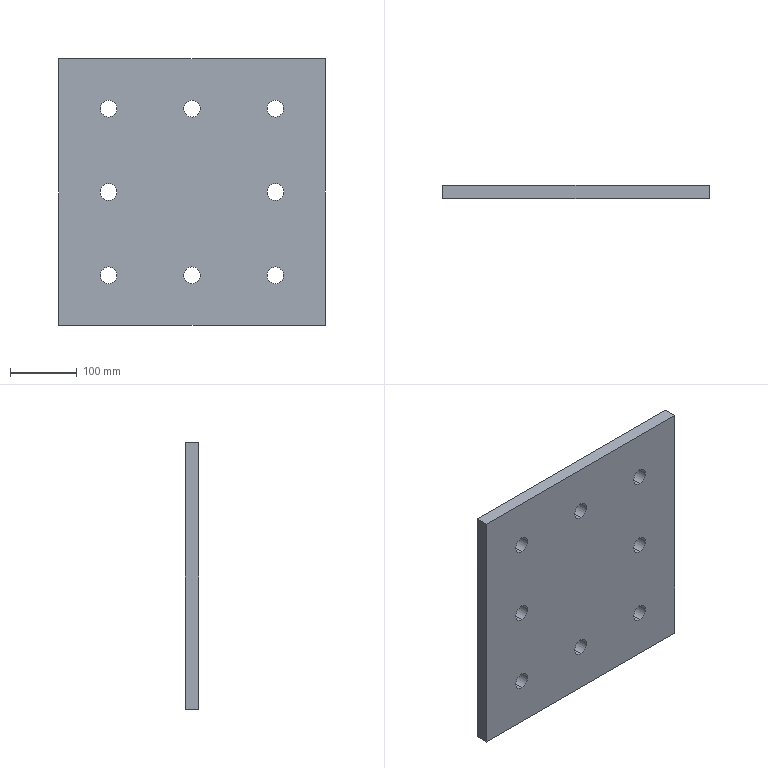Component | SolidWorks | SmallFlange20-5 | 1 solid | 22 faces | box 400 x 20 x 400 mm | volume 3121460 mm3 | cylinder 16 | plane 6 | commonest cylinder face diameters 25 x16 | material Plain Carbon Steel
STEP:
#1=COLOUR_RGB('',0.7922,0.8196,0.9333);
#2=FILL_AREA_STYLE_COLOUR('',#1);
#3=FILL_AREA_STYLE('',(#2));
#4=SURFACE_STYLE_FILL_AREA(#3);
#5=SURFACE_SIDE_STYLE('',(#4));
#6=SURFACE_STYLE_USAGE(.BOTH.,#5);
#7=PRESENTATION_STYLE_ASSIGNMENT((#6));
#8=CARTESIAN_POINT('',(668.501,114.165,68.614));
#9=VERTEX_POINT('',#8);
#10=CARTESIAN_POINT('',(668.501,114.165,67.629));
#11=VERTEX_POINT('',#10);
#12=CARTESIAN_POINT('',(668.501,114.165,68.122));
#13=DIRECTION('',(0.,1.,-0.));
#14=DIRECTION('',(0.,0.,-1.));
#15=AXIS2_PLACEMENT_3D('',#12,#13,#14);
#16=CIRCLE('',#15,0.4921);
#17=EDGE_CURVE('',#9,#11,#16,.T.);
#18=ORIENTED_EDGE('',*,*,#17,.F.);
#19=CARTESIAN_POINT('',(668.501,114.953,68.614));
#20=VERTEX_POINT('',#19);
#21=CARTESIAN_POINT('',(668.501,114.165,68.614));
#22=DIRECTION('',(0.,1.,-0.));
#23=VECTOR('',#22,39.37);
#24=LINE('',#21,#23);
#25=EDGE_CURVE('',#9,#20,#24,.T.);
#26=ORIENTED_EDGE('',*,*,#25,.T.);
#27=CARTESIAN_POINT('',(668.501,114.953,67.629));
#28=VERTEX_POINT('',#27);
#29=CARTESIAN_POINT('',(668.501,114.953,68.122));
#30=DIRECTION('',(0.,1.,-0.));
#31=DIRECTION('',(0.,0.,-1.));
#32=AXIS2_PLACEMENT_3D('',#29,#30,#31);
#33=CIRCLE('',#32,0.4921);
#34=EDGE_CURVE('',#20,#28,#33,.T.);
#35=ORIENTED_EDGE('',*,*,#34,.T.);
#36=CARTESIAN_POINT('',(668.501,114.165,67.629));
#37=DIRECTION('',(0.,1.,-0.));
#38=VECTOR('',#37,39.37);
#39=LINE('',#36,#38);
#40=EDGE_CURVE('',#11,#28,#39,.T.);
#41=ORIENTED_EDGE('',*,*,#40,.F.);
#42=EDGE_LOOP('',(#18,#26,#35,#41));
#43=FACE_OUTER_BOUND('',#42,.T.);
#44=CARTESIAN_POINT('',(668.501,114.165,68.122));
#45=DIRECTION('',(0.,1.,-0.));
#46=DIRECTION('',(0.,0.,-1.));
#47=AXIS2_PLACEMENT_3D('',#44,#45,#46);
#48=CYLINDRICAL_SURFACE('',#47,0.4921);
#49=ADVANCED_FACE('',(#43),#48,.F.);
#50=CARTESIAN_POINT('',(668.501,114.165,73.535));
#51=VERTEX_POINT('',#50);
#52=CARTESIAN_POINT('',(668.501,114.165,72.551));
#53=VERTEX_POINT('',#52);
#54=CARTESIAN_POINT('',(668.501,114.165,73.043));
#55=DIRECTION('',(0.,1.,-0.));
#56=DIRECTION('',(0.,0.,-1.));
#57=AXIS2_PLACEMENT_3D('',#54,#55,#56);
#58=CIRCLE('',#57,0.4921);
#59=EDGE_CURVE('',#51,#53,#58,.T.);
#60=ORIENTED_EDGE('',*,*,#59,.F.);
#61=CARTESIAN_POINT('',(668.501,114.953,73.535));
#62=VERTEX_POINT('',#61);
#63=CARTESIAN_POINT('',(668.501,114.165,73.535));
#64=DIRECTION('',(0.,1.,-0.));
#65=VECTOR('',#64,39.37);
#66=LINE('',#63,#65);
#67=EDGE_CURVE('',#51,#62,#66,.T.);
#68=ORIENTED_EDGE('',*,*,#67,.T.);
#69=CARTESIAN_POINT('',(668.501,114.953,72.551));
#70=VERTEX_POINT('',#69);
#71=CARTESIAN_POINT('',(668.501,114.953,73.043));
#72=DIRECTION('',(0.,1.,-0.));
#73=DIRECTION('',(0.,0.,-1.));
#74=AXIS2_PLACEMENT_3D('',#71,#72,#73);
#75=CIRCLE('',#74,0.4921);
#76=EDGE_CURVE('',#62,#70,#75,.T.);
#77=ORIENTED_EDGE('',*,*,#76,.T.);
#78=CARTESIAN_POINT('',(668.501,114.165,72.551));
#79=DIRECTION('',(0.,1.,-0.));
#80=VECTOR('',#79,39.37);
#81=LINE('',#78,#80);
#82=EDGE_CURVE('',#53,#70,#81,.T.);
#83=ORIENTED_EDGE('',*,*,#82,.F.);
#84=EDGE_LOOP('',(#60,#68,#77,#83));
#85=FACE_OUTER_BOUND('',#84,.T.);
#86=CARTESIAN_POINT('',(668.501,114.165,73.043));
#87=DIRECTION('',(0.,1.,-0.));
#88=DIRECTION('',(0.,0.,-1.));
#89=AXIS2_PLACEMENT_3D('',#86,#87,#88);
#90=CYLINDRICAL_SURFACE('',#89,0.4921);
#91=ADVANCED_FACE('',(#85),#90,.F.);
#92=CARTESIAN_POINT('',(658.659,114.165,68.614));
#93=VERTEX_POINT('',#92);
#94=CARTESIAN_POINT('',(658.659,114.165,67.629));
#95=VERTEX_POINT('',#94);
#96=CARTESIAN_POINT('',(658.659,114.165,68.122));
#97=DIRECTION('',(0.,1.,-0.));
#98=DIRECTION('',(0.,0.,-1.));
#99=AXIS2_PLACEMENT_3D('',#96,#97,#98);
#100=CIRCLE('',#99,0.4921);
#101=EDGE_CURVE('',#93,#95,#100,.T.);
#102=ORIENTED_EDGE('',*,*,#101,.F.);
#103=CARTESIAN_POINT('',(658.659,114.953,68.614));
#104=VERTEX_POINT('',#103);
#105=CARTESIAN_POINT('',(658.659,114.165,68.614));
#106=DIRECTION('',(0.,1.,-0.));
#107=VECTOR('',#106,39.37);
#108=LINE('',#105,#107);
#109=EDGE_CURVE('',#93,#104,#108,.T.);
#110=ORIENTED_EDGE('',*,*,#109,.T.);
#111=CARTESIAN_POINT('',(658.659,114.953,67.629));
#112=VERTEX_POINT('',#111);
#113=CARTESIAN_POINT('',(658.659,114.953,68.122));
#114=DIRECTION('',(0.,1.,-0.));
#115=DIRECTION('',(0.,0.,-1.));
#116=AXIS2_PLACEMENT_3D('',#113,#114,#115);
#117=CIRCLE('',#116,0.4921);
#118=EDGE_CURVE('',#104,#112,#117,.T.);
#119=ORIENTED_EDGE('',*,*,#118,.T.);
#120=CARTESIAN_POINT('',(658.659,114.165,67.629));
#121=DIRECTION('',(0.,1.,-0.));
#122=VECTOR('',#121,39.37);
#123=LINE('',#120,#122);
#124=EDGE_CURVE('',#95,#112,#123,.T.);
#125=ORIENTED_EDGE('',*,*,#124,.F.);
#126=EDGE_LOOP('',(#102,#110,#119,#125));
#127=FACE_OUTER_BOUND('',#126,.T.);
#128=CARTESIAN_POINT('',(658.659,114.165,68.122));
#129=DIRECTION('',(0.,1.,-0.));
#130=DIRECTION('',(0.,0.,-1.));
#131=AXIS2_PLACEMENT_3D('',#128,#129,#130);
#132=CYLINDRICAL_SURFACE('',#131,0.4921);
#133=ADVANCED_FACE('',(#127),#132,.F.);
#134=CARTESIAN_POINT('',(663.58,114.165,68.614));
#135=VERTEX_POINT('',#134);
#136=CARTESIAN_POINT('',(663.58,114.165,67.629));
#137=VERTEX_POINT('',#136);
#138=CARTESIAN_POINT('',(663.58,114.165,68.122));
#139=DIRECTION('',(0.,1.,-0.));
#140=DIRECTION('',(0.,0.,-1.));
#141=AXIS2_PLACEMENT_3D('',#138,#139,#140);
#142=CIRCLE('',#141,0.4921);
#143=EDGE_CURVE('',#135,#137,#142,.T.);
#144=ORIENTED_EDGE('',*,*,#143,.F.);
#145=CARTESIAN_POINT('',(663.58,114.953,68.614));
#146=VERTEX_POINT('',#145);
#147=CARTESIAN_POINT('',(663.58,114.165,68.614));
#148=DIRECTION('',(0.,1.,-0.));
#149=VECTOR('',#148,39.37);
#150=LINE('',#147,#149);
#151=EDGE_CURVE('',#135,#146,#150,.T.);
#152=ORIENTED_EDGE('',*,*,#151,.T.);
#153=CARTESIAN_POINT('',(663.58,114.953,67.629));
#154=VERTEX_POINT('',#153);
#155=CARTESIAN_POINT('',(663.58,114.953,68.122));
#156=DIRECTION('',(0.,1.,-0.));
#157=DIRECTION('',(0.,0.,-1.));
#158=AXIS2_PLACEMENT_3D('',#155,#156,#157);
#159=CIRCLE('',#158,0.4921);
#160=EDGE_CURVE('',#146,#154,#159,.T.);
#161=ORIENTED_EDGE('',*,*,#160,.T.);
#162=CARTESIAN_POINT('',(663.58,114.165,67.629));
#163=DIRECTION('',(0.,1.,-0.));
#164=VECTOR('',#163,39.37);
#165=LINE('',#162,#164);
#166=EDGE_CURVE('',#137,#154,#165,.T.);
#167=ORIENTED_EDGE('',*,*,#166,.F.);
#168=EDGE_LOOP('',(#144,#152,#161,#167));
#169=FACE_OUTER_BOUND('',#168,.T.);
#170=CARTESIAN_POINT('',(663.58,114.165,68.122));
#171=DIRECTION('',(0.,1.,-0.));
#172=DIRECTION('',(0.,0.,-1.));
#173=AXIS2_PLACEMENT_3D('',#170,#171,#172);
#174=CYLINDRICAL_SURFACE('',#173,0.4921);
#175=ADVANCED_FACE('',(#169),#174,.F.);
#176=CARTESIAN_POINT('',(658.659,114.165,73.535));
#177=VERTEX_POINT('',#176);
#178=CARTESIAN_POINT('',(658.659,114.165,72.551));
#179=VERTEX_POINT('',#178);
#180=CARTESIAN_POINT('',(658.659,114.165,73.043));
#181=DIRECTION('',(0.,1.,-0.));
#182=DIRECTION('',(0.,0.,-1.));
#183=AXIS2_PLACEMENT_3D('',#180,#181,#182);
#184=CIRCLE('',#183,0.4921);
#185=EDGE_CURVE('',#177,#179,#184,.T.);
#186=ORIENTED_EDGE('',*,*,#185,.F.);
#187=CARTESIAN_POINT('',(658.659,114.953,73.535));
#188=VERTEX_POINT('',#187);
#189=CARTESIAN_POINT('',(658.659,114.165,73.535));
#190=DIRECTION('',(0.,1.,-0.));
#191=VECTOR('',#190,39.37);
#192=LINE('',#189,#191);
#193=EDGE_CURVE('',#177,#188,#192,.T.);
#194=ORIENTED_EDGE('',*,*,#193,.T.);
#195=CARTESIAN_POINT('',(658.659,114.953,72.551));
#196=VERTEX_POINT('',#195);
#197=CARTESIAN_POINT('',(658.659,114.953,73.043));
#198=DIRECTION('',(0.,1.,-0.));
#199=DIRECTION('',(0.,0.,-1.));
#200=AXIS2_PLACEMENT_3D('',#197,#198,#199);
#201=CIRCLE('',#200,0.4921);
#202=EDGE_CURVE('',#188,#196,#201,.T.);
#203=ORIENTED_EDGE('',*,*,#202,.T.);
#204=CARTESIAN_POINT('',(658.659,114.165,72.551));
#205=DIRECTION('',(0.,1.,-0.));
#206=VECTOR('',#205,39.37);
#207=LINE('',#204,#206);
#208=EDGE_CURVE('',#179,#196,#207,.T.);
#209=ORIENTED_EDGE('',*,*,#208,.F.);
#210=EDGE_LOOP('',(#186,#194,#203,#209));
#211=FACE_OUTER_BOUND('',#210,.T.);
#212=CARTESIAN_POINT('',(658.659,114.165,73.043));
#213=DIRECTION('',(0.,1.,-0.));
#214=DIRECTION('',(0.,0.,-1.));
#215=AXIS2_PLACEMENT_3D('',#212,#213,#214);
#216=CYLINDRICAL_SURFACE('',#215,0.4921);
#217=ADVANCED_FACE('',(#211),#216,.F.);
#218=CARTESIAN_POINT('',(658.659,114.165,78.456));
#219=VERTEX_POINT('',#218);
#220=CARTESIAN_POINT('',(658.659,114.165,77.472));
#221=VERTEX_POINT('',#220);
#222=CARTESIAN_POINT('',(658.659,114.165,77.964));
#223=DIRECTION('',(0.,1.,-0.));
#224=DIRECTION('',(0.,0.,-1.));
#225=AXIS2_PLACEMENT_3D('',#222,#223,#224);
#226=CIRCLE('',#225,0.4921);
#227=EDGE_CURVE('',#219,#221,#226,.T.);
#228=ORIENTED_EDGE('',*,*,#227,.F.);
#229=CARTESIAN_POINT('',(658.659,114.953,78.456));
#230=VERTEX_POINT('',#229);
#231=CARTESIAN_POINT('',(658.659,114.165,78.456));
#232=DIRECTION('',(0.,1.,-0.));
#233=VECTOR('',#232,39.37);
#234=LINE('',#231,#233);
#235=EDGE_CURVE('',#219,#230,#234,.T.);
#236=ORIENTED_EDGE('',*,*,#235,.T.);
#237=CARTESIAN_POINT('',(658.659,114.953,77.472));
#238=VERTEX_POINT('',#237);
#239=CARTESIAN_POINT('',(658.659,114.953,77.964));
#240=DIRECTION('',(0.,1.,-0.));
#241=DIRECTION('',(0.,0.,-1.));
#242=AXIS2_PLACEMENT_3D('',#239,#240,#241);
#243=CIRCLE('',#242,0.4921);
#244=EDGE_CURVE('',#230,#238,#243,.T.);
#245=ORIENTED_EDGE('',*,*,#244,.T.);
#246=CARTESIAN_POINT('',(658.659,114.165,77.472));
#247=DIRECTION('',(0.,1.,-0.));
#248=VECTOR('',#247,39.37);
#249=LINE('',#246,#248);
#250=EDGE_CURVE('',#221,#238,#249,.T.);
#251=ORIENTED_EDGE('',*,*,#250,.F.);
#252=EDGE_LOOP('',(#228,#236,#245,#251));
#253=FACE_OUTER_BOUND('',#252,.T.);
#254=CARTESIAN_POINT('',(658.659,114.165,77.964));
#255=DIRECTION('',(0.,1.,-0.));
#256=DIRECTION('',(0.,0.,-1.));
#257=AXIS2_PLACEMENT_3D('',#254,#255,#256);
#258=CYLINDRICAL_SURFACE('',#257,0.4921);
#259=ADVANCED_FACE('',(#253),#258,.F.);
#260=CARTESIAN_POINT('',(663.58,114.165,78.456));
#261=VERTEX_POINT('',#260);
#262=CARTESIAN_POINT('',(663.58,114.165,77.472));
#263=VERTEX_POINT('',#262);
#264=CARTESIAN_POINT('',(663.58,114.165,77.964));
#265=DIRECTION('',(0.,1.,-0.));
#266=DIRECTION('',(0.,0.,-1.));
#267=AXIS2_PLACEMENT_3D('',#264,#265,#266);
#268=CIRCLE('',#267,0.4921);
#269=EDGE_CURVE('',#261,#263,#268,.T.);
#270=ORIENTED_EDGE('',*,*,#269,.F.);
#271=CARTESIAN_POINT('',(663.58,114.953,78.456));
#272=VERTEX_POINT('',#271);
#273=CARTESIAN_POINT('',(663.58,114.165,78.456));
#274=DIRECTION('',(0.,1.,-0.));
#275=VECTOR('',#274,39.37);
#276=LINE('',#273,#275);
#277=EDGE_CURVE('',#261,#272,#276,.T.);
#278=ORIENTED_EDGE('',*,*,#277,.T.);
#279=CARTESIAN_POINT('',(663.58,114.953,77.472));
#280=VERTEX_POINT('',#279);
#281=CARTESIAN_POINT('',(663.58,114.953,77.964));
#282=DIRECTION('',(0.,1.,-0.));
#283=DIRECTION('',(0.,0.,-1.));
#284=AXIS2_PLACEMENT_3D('',#281,#282,#283);
#285=CIRCLE('',#284,0.4921);
#286=EDGE_CURVE('',#272,#280,#285,.T.);
#287=ORIENTED_EDGE('',*,*,#286,.T.);
#288=CARTESIAN_POINT('',(663.58,114.165,77.472));
#289=DIRECTION('',(0.,1.,-0.));
#290=VECTOR('',#289,39.37);
#291=LINE('',#288,#290);
#292=EDGE_CURVE('',#263,#280,#291,.T.);
#293=ORIENTED_EDGE('',*,*,#292,.F.);
#294=EDGE_LOOP('',(#270,#278,#287,#293));
#295=FACE_OUTER_BOUND('',#294,.T.);
#296=CARTESIAN_POINT('',(663.58,114.165,77.964));
#297=DIRECTION('',(0.,1.,-0.));
#298=DIRECTION('',(0.,0.,-1.));
#299=AXIS2_PLACEMENT_3D('',#296,#297,#298);
#300=CYLINDRICAL_SURFACE('',#299,0.4921);
#301=ADVANCED_FACE('',(#295),#300,.F.);
#302=CARTESIAN_POINT('',(668.501,114.165,78.456));
#303=VERTEX_POINT('',#302);
#304=CARTESIAN_POINT('',(668.501,114.165,77.472));
#305=VERTEX_POINT('',#304);
#306=CARTESIAN_POINT('',(668.501,114.165,77.964));
#307=DIRECTION('',(0.,1.,-0.));
#308=DIRECTION('',(0.,0.,-1.));
#309=AXIS2_PLACEMENT_3D('',#306,#307,#308);
#310=CIRCLE('',#309,0.4921);
#311=EDGE_CURVE('',#303,#305,#310,.T.);
#312=ORIENTED_EDGE('',*,*,#311,.F.);
#313=CARTESIAN_POINT('',(668.501,114.953,78.456));
#314=VERTEX_POINT('',#313);
#315=CARTESIAN_POINT('',(668.501,114.165,78.456));
#316=DIRECTION('',(0.,1.,-0.));
#317=VECTOR('',#316,39.37);
#318=LINE('',#315,#317);
#319=EDGE_CURVE('',#303,#314,#318,.T.);
#320=ORIENTED_EDGE('',*,*,#319,.T.);
#321=CARTESIAN_POINT('',(668.501,114.953,77.472));
#322=VERTEX_POINT('',#321);
#323=CARTESIAN_POINT('',(668.501,114.953,77.964));
#324=DIRECTION('',(0.,1.,-0.));
#325=DIRECTION('',(0.,0.,-1.));
#326=AXIS2_PLACEMENT_3D('',#323,#324,#325);
#327=CIRCLE('',#326,0.4921);
#328=EDGE_CURVE('',#314,#322,#327,.T.);
#329=ORIENTED_EDGE('',*,*,#328,.T.);
#330=CARTESIAN_POINT('',(668.501,114.165,77.472));
#331=DIRECTION('',(0.,1.,-0.));
#332=VECTOR('',#331,39.37);
#333=LINE('',#330,#332);
#334=EDGE_CURVE('',#305,#322,#333,.T.);
#335=ORIENTED_EDGE('',*,*,#334,.F.);
#336=EDGE_LOOP('',(#312,#320,#329,#335));
#337=FACE_OUTER_BOUND('',#336,.T.);
#338=CARTESIAN_POINT('',(668.501,114.165,77.964));
#339=DIRECTION('',(0.,1.,-0.));
#340=DIRECTION('',(0.,0.,-1.));
#341=AXIS2_PLACEMENT_3D('',#338,#339,#340);
#342=CYLINDRICAL_SURFACE('',#341,0.4921);
#343=ADVANCED_FACE('',(#337),#342,.F.);
#344=CARTESIAN_POINT('',(655.706,114.953,65.169));
#345=VERTEX_POINT('',#344);
#346=CARTESIAN_POINT('',(655.706,114.953,80.917));
#347=VERTEX_POINT('',#346);
#348=CARTESIAN_POINT('',(655.706,114.953,80.917));
#349=DIRECTION('',(0.,-0.,1.));
#350=VECTOR('',#349,39.37);
#351=LINE('',#348,#350);
#352=EDGE_CURVE('',#345,#347,#351,.T.);
#353=ORIENTED_EDGE('',*,*,#352,.F.);
#354=CARTESIAN_POINT('',(655.706,114.165,65.169));
#355=VERTEX_POINT('',#354);
#356=CARTESIAN_POINT('',(655.706,114.165,65.169));
#357=DIRECTION('',(0.,1.,-0.));
#358=VECTOR('',#357,39.37);
#359=LINE('',#356,#358);
#360=EDGE_CURVE('',#355,#345,#359,.T.);
#361=ORIENTED_EDGE('',*,*,#360,.F.);
#362=CARTESIAN_POINT('',(655.706,114.165,80.917));
#363=VERTEX_POINT('',#362);
#364=CARTESIAN_POINT('',(655.706,114.165,80.917));
#365=DIRECTION('',(0.,-0.,1.));
#366=VECTOR('',#365,39.37);
#367=LINE('',#364,#366);
#368=EDGE_CURVE('',#355,#363,#367,.T.);
#369=ORIENTED_EDGE('',*,*,#368,.T.);
#370=CARTESIAN_POINT('',(655.706,114.165,80.917));
#371=DIRECTION('',(0.,1.,-0.));
#372=VECTOR('',#371,39.37);
#373=LINE('',#370,#372);
#374=EDGE_CURVE('',#363,#347,#373,.T.);
#375=ORIENTED_EDGE('',*,*,#374,.T.);
#376=EDGE_LOOP('',(#353,#361,#369,#375));
#377=FACE_OUTER_BOUND('',#376,.T.);
#378=CARTESIAN_POINT('',(655.706,114.165,80.917));
#379=DIRECTION('',(-1.,0.,0.));
#380=DIRECTION('',(0.,-0.,1.));
#381=AXIS2_PLACEMENT_3D('',#378,#379,#380);
#382=PLANE('',#381);
#383=ADVANCED_FACE('',(#377),#382,.T.);
#384=CARTESIAN_POINT('',(671.454,114.953,65.169));
#385=VERTEX_POINT('',#384);
#386=CARTESIAN_POINT('',(671.454,114.953,65.169));
#387=DIRECTION('',(-1.,0.,0.));
#388=VECTOR('',#387,39.37);
#389=LINE('',#386,#388);
#390=EDGE_CURVE('',#385,#345,#389,.T.);
#391=ORIENTED_EDGE('',*,*,#390,.F.);
#392=CARTESIAN_POINT('',(671.454,114.165,65.169));
#393=VERTEX_POINT('',#392);
#394=CARTESIAN_POINT('',(671.454,114.165,65.169));
#395=DIRECTION('',(0.,1.,-0.));
#396=VECTOR('',#395,39.37);
#397=LINE('',#394,#396);
#398=EDGE_CURVE('',#393,#385,#397,.T.);
#399=ORIENTED_EDGE('',*,*,#398,.F.);
#400=CARTESIAN_POINT('',(671.454,114.165,65.169));
#401=DIRECTION('',(-1.,0.,0.));
#402=VECTOR('',#401,39.37);
#403=LINE('',#400,#402);
#404=EDGE_CURVE('',#393,#355,#403,.T.);
#405=ORIENTED_EDGE('',*,*,#404,.T.);
#406=ORIENTED_EDGE('',*,*,#360,.T.);
#407=EDGE_LOOP('',(#391,#399,#405,#406));
#408=FACE_OUTER_BOUND('',#407,.T.);
#409=CARTESIAN_POINT('',(671.454,114.165,65.169));
#410=DIRECTION('',(-0.,0.,-1.));
#411=DIRECTION('',(-1.,0.,0.));
#412=AXIS2_PLACEMENT_3D('',#409,#410,#411);
#413=PLANE('',#412);
#414=ADVANCED_FACE('',(#408),#413,.T.);
#415=CARTESIAN_POINT('',(671.454,114.953,80.917));
#416=VERTEX_POINT('',#415);
#417=CARTESIAN_POINT('',(671.454,114.953,80.917));
#418=DIRECTION('',(-0.,0.,-1.));
#419=VECTOR('',#418,39.37);
#420=LINE('',#417,#419);
#421=EDGE_CURVE('',#416,#385,#420,.T.);
#422=ORIENTED_EDGE('',*,*,#421,.F.);
#423=CARTESIAN_POINT('',(671.454,114.165,80.917));
#424=VERTEX_POINT('',#423);
#425=CARTESIAN_POINT('',(671.454,114.165,80.917));
#426=DIRECTION('',(0.,1.,-0.));
#427=VECTOR('',#426,39.37);
#428=LINE('',#425,#427);
#429=EDGE_CURVE('',#424,#416,#428,.T.);
#430=ORIENTED_EDGE('',*,*,#429,.F.);
#431=CARTESIAN_POINT('',(671.454,114.165,80.917));
#432=DIRECTION('',(-0.,0.,-1.));
#433=VECTOR('',#432,39.37);
#434=LINE('',#431,#433);
#435=EDGE_CURVE('',#424,#393,#434,.T.);
#436=ORIENTED_EDGE('',*,*,#435,.T.);
#437=ORIENTED_EDGE('',*,*,#398,.T.);
#438=EDGE_LOOP('',(#422,#430,#436,#437));
#439=FACE_OUTER_BOUND('',#438,.T.);
#440=CARTESIAN_POINT('',(671.454,114.165,80.917));
#441=DIRECTION('',(1.,-0.,-0.));
#442=DIRECTION('',(-0.,0.,-1.));
#443=AXIS2_PLACEMENT_3D('',#440,#441,#442);
#444=PLANE('',#443);
#445=ADVANCED_FACE('',(#439),#444,.T.);
#446=CARTESIAN_POINT('',(671.454,114.953,80.917));
#447=DIRECTION('',(1.,-0.,-0.));
#448=VECTOR('',#447,39.37);
#449=LINE('',#446,#448);
#450=EDGE_CURVE('',#347,#416,#449,.T.);
#451=ORIENTED_EDGE('',*,*,#450,.F.);
#452=ORIENTED_EDGE('',*,*,#374,.F.);
#453=CARTESIAN_POINT('',(671.454,114.165,80.917));
#454=DIRECTION('',(1.,-0.,-0.));
#455=VECTOR('',#454,39.37);
#456=LINE('',#453,#455);
#457=EDGE_CURVE('',#363,#424,#456,.T.);
#458=ORIENTED_EDGE('',*,*,#457,.T.);
#459=ORIENTED_EDGE('',*,*,#429,.T.);
#460=EDGE_LOOP('',(#451,#452,#458,#459));
#461=FACE_OUTER_BOUND('',#460,.T.);
#462=CARTESIAN_POINT('',(671.454,114.165,80.917));
#463=DIRECTION('',(0.,-0.,1.));
#464=DIRECTION('',(1.,-0.,-0.));
#465=AXIS2_PLACEMENT_3D('',#462,#463,#464);
#466=PLANE('',#465);
#467=ADVANCED_FACE('',(#461),#466,.T.);
#468=CARTESIAN_POINT('',(668.501,114.165,68.122));
#469=DIRECTION('',(0.,1.,-0.));
#470=DIRECTION('',(0.,0.,-1.));
#471=AXIS2_PLACEMENT_3D('',#468,#469,#470);
#472=CIRCLE('',#471,0.4921);
#473=EDGE_CURVE('',#11,#9,#472,.T.);
#474=ORIENTED_EDGE('',*,*,#473,.T.);
#475=ORIENTED_EDGE('',*,*,#17,.T.);
#476=EDGE_LOOP('',(#474,#475));
#477=FACE_BOUND('',#476,.T.);
#478=CARTESIAN_POINT('',(668.501,114.165,73.043));
#479=DIRECTION('',(0.,1.,-0.));
#480=DIRECTION('',(0.,0.,-1.));
#481=AXIS2_PLACEMENT_3D('',#478,#479,#480);
#482=CIRCLE('',#481,0.4921);
#483=EDGE_CURVE('',#53,#51,#482,.T.);
#484=ORIENTED_EDGE('',*,*,#483,.T.);
#485=ORIENTED_EDGE('',*,*,#59,.T.);
#486=EDGE_LOOP('',(#484,#485));
#487=FACE_BOUND('',#486,.T.);
#488=CARTESIAN_POINT('',(658.659,114.165,68.122));
#489=DIRECTION('',(0.,1.,-0.));
#490=DIRECTION('',(0.,0.,-1.));
#491=AXIS2_PLACEMENT_3D('',#488,#489,#490);
#492=CIRCLE('',#491,0.4921);
#493=EDGE_CURVE('',#95,#93,#492,.T.);
#494=ORIENTED_EDGE('',*,*,#493,.T.);
#495=ORIENTED_EDGE('',*,*,#101,.T.);
#496=EDGE_LOOP('',(#494,#495));
#497=FACE_BOUND('',#496,.T.);
#498=CARTESIAN_POINT('',(663.58,114.165,68.122));
#499=DIRECTION('',(0.,1.,-0.));
#500=DIRECTION('',(0.,0.,-1.));
#501=AXIS2_PLACEMENT_3D('',#498,#499,#500);
#502=CIRCLE('',#501,0.4921);
#503=EDGE_CURVE('',#137,#135,#502,.T.);
#504=ORIENTED_EDGE('',*,*,#503,.T.);
#505=ORIENTED_EDGE('',*,*,#143,.T.);
#506=EDGE_LOOP('',(#504,#505));
#507=FACE_BOUND('',#506,.T.);
#508=CARTESIAN_POINT('',(658.659,114.165,73.043));
#509=DIRECTION('',(0.,1.,-0.));
#510=DIRECTION('',(0.,0.,-1.));
#511=AXIS2_PLACEMENT_3D('',#508,#509,#510);
#512=CIRCLE('',#511,0.4921);
#513=EDGE_CURVE('',#179,#177,#512,.T.);
#514=ORIENTED_EDGE('',*,*,#513,.T.);
#515=ORIENTED_EDGE('',*,*,#185,.T.);
#516=EDGE_LOOP('',(#514,#515));
#517=FACE_BOUND('',#516,.T.);
#518=CARTESIAN_POINT('',(658.659,114.165,77.964));
#519=DIRECTION('',(0.,1.,-0.));
#520=DIRECTION('',(0.,0.,-1.));
#521=AXIS2_PLACEMENT_3D('',#518,#519,#520);
#522=CIRCLE('',#521,0.4921);
#523=EDGE_CURVE('',#221,#219,#522,.T.);
#524=ORIENTED_EDGE('',*,*,#523,.T.);
#525=ORIENTED_EDGE('',*,*,#227,.T.);
#526=EDGE_LOOP('',(#524,#525));
#527=FACE_BOUND('',#526,.T.);
#528=CARTESIAN_POINT('',(663.58,114.165,77.964));
#529=DIRECTION('',(0.,1.,-0.));
#530=DIRECTION('',(0.,0.,-1.));
#531=AXIS2_PLACEMENT_3D('',#528,#529,#530);
#532=CIRCLE('',#531,0.4921);
#533=EDGE_CURVE('',#263,#261,#532,.T.);
#534=ORIENTED_EDGE('',*,*,#533,.T.);
#535=ORIENTED_EDGE('',*,*,#269,.T.);
#536=EDGE_LOOP('',(#534,#535));
#537=FACE_BOUND('',#536,.T.);
#538=CARTESIAN_POINT('',(668.501,114.165,77.964));
#539=DIRECTION('',(0.,1.,-0.));
#540=DIRECTION('',(0.,0.,-1.));
#541=AXIS2_PLACEMENT_3D('',#538,#539,#540);
#542=CIRCLE('',#541,0.4921);
#543=EDGE_CURVE('',#305,#303,#542,.T.);
#544=ORIENTED_EDGE('',*,*,#543,.T.);
#545=ORIENTED_EDGE('',*,*,#311,.T.);
#546=EDGE_LOOP('',(#544,#545));
#547=FACE_BOUND('',#546,.T.);
#548=ORIENTED_EDGE('',*,*,#368,.F.);
#549=ORIENTED_EDGE('',*,*,#404,.F.);
#550=ORIENTED_EDGE('',*,*,#435,.F.);
#551=ORIENTED_EDGE('',*,*,#457,.F.);
#552=EDGE_LOOP('',(#548,#549,#550,#551));
#553=FACE_OUTER_BOUND('',#552,.T.);
#554=CARTESIAN_POINT('',(663.58,114.165,73.043));
#555=DIRECTION('',(0.,1.,-0.));
#556=DIRECTION('',(-0.,0.,-1.));
#557=AXIS2_PLACEMENT_3D('',#554,#555,#556);
#558=PLANE('',#557);
#559=ADVANCED_FACE('',(#477,#487,#497,#507,#517,#527,#537,#547,#553),#558,.F.);
#560=CARTESIAN_POINT('',(668.501,114.953,68.122));
#561=DIRECTION('',(0.,1.,-0.));
#562=DIRECTION('',(0.,0.,-1.));
#563=AXIS2_PLACEMENT_3D('',#560,#561,#562);
#564=CIRCLE('',#563,0.4921);
#565=EDGE_CURVE('',#28,#20,#564,.T.);
#566=ORIENTED_EDGE('',*,*,#565,.F.);
#567=ORIENTED_EDGE('',*,*,#34,.F.);
#568=EDGE_LOOP('',(#566,#567));
#569=FACE_BOUND('',#568,.T.);
#570=CARTESIAN_POINT('',(668.501,114.953,73.043));
#571=DIRECTION('',(0.,1.,-0.));
#572=DIRECTION('',(0.,0.,-1.));
#573=AXIS2_PLACEMENT_3D('',#570,#571,#572);
#574=CIRCLE('',#573,0.4921);
#575=EDGE_CURVE('',#70,#62,#574,.T.);
#576=ORIENTED_EDGE('',*,*,#575,.F.);
#577=ORIENTED_EDGE('',*,*,#76,.F.);
#578=EDGE_LOOP('',(#576,#577));
#579=FACE_BOUND('',#578,.T.);
#580=CARTESIAN_POINT('',(658.659,114.953,68.122));
#581=DIRECTION('',(0.,1.,-0.));
#582=DIRECTION('',(0.,0.,-1.));
#583=AXIS2_PLACEMENT_3D('',#580,#581,#582);
#584=CIRCLE('',#583,0.4921);
#585=EDGE_CURVE('',#112,#104,#584,.T.);
#586=ORIENTED_EDGE('',*,*,#585,.F.);
#587=ORIENTED_EDGE('',*,*,#118,.F.);
#588=EDGE_LOOP('',(#586,#587));
#589=FACE_BOUND('',#588,.T.);
#590=CARTESIAN_POINT('',(663.58,114.953,68.122));
#591=DIRECTION('',(0.,1.,-0.));
#592=DIRECTION('',(0.,0.,-1.));
#593=AXIS2_PLACEMENT_3D('',#590,#591,#592);
#594=CIRCLE('',#593,0.4921);
#595=EDGE_CURVE('',#154,#146,#594,.T.);
#596=ORIENTED_EDGE('',*,*,#595,.F.);
#597=ORIENTED_EDGE('',*,*,#160,.F.);
#598=EDGE_LOOP('',(#596,#597));
#599=FACE_BOUND('',#598,.T.);
#600=CARTESIAN_POINT('',(658.659,114.953,73.043));
#601=DIRECTION('',(0.,1.,-0.));
#602=DIRECTION('',(0.,0.,-1.));
#603=AXIS2_PLACEMENT_3D('',#600,#601,#602);
#604=CIRCLE('',#603,0.4921);
#605=EDGE_CURVE('',#196,#188,#604,.T.);
#606=ORIENTED_EDGE('',*,*,#605,.F.);
#607=ORIENTED_EDGE('',*,*,#202,.F.);
#608=EDGE_LOOP('',(#606,#607));
#609=FACE_BOUND('',#608,.T.);
#610=CARTESIAN_POINT('',(658.659,114.953,77.964));
#611=DIRECTION('',(0.,1.,-0.));
#612=DIRECTION('',(0.,0.,-1.));
#613=AXIS2_PLACEMENT_3D('',#610,#611,#612);
#614=CIRCLE('',#613,0.4921);
#615=EDGE_CURVE('',#238,#230,#614,.T.);
#616=ORIENTED_EDGE('',*,*,#615,.F.);
#617=ORIENTED_EDGE('',*,*,#244,.F.);
#618=EDGE_LOOP('',(#616,#617));
#619=FACE_BOUND('',#618,.T.);
#620=CARTESIAN_POINT('',(663.58,114.953,77.964));
#621=DIRECTION('',(0.,1.,-0.));
#622=DIRECTION('',(0.,0.,-1.));
#623=AXIS2_PLACEMENT_3D('',#620,#621,#622);
#624=CIRCLE('',#623,0.4921);
#625=EDGE_CURVE('',#280,#272,#624,.T.);
#626=ORIENTED_EDGE('',*,*,#625,.F.);
#627=ORIENTED_EDGE('',*,*,#286,.F.);
#628=EDGE_LOOP('',(#626,#627));
#629=FACE_BOUND('',#628,.T.);
#630=CARTESIAN_POINT('',(668.501,114.953,77.964));
#631=DIRECTION('',(0.,1.,-0.));
#632=DIRECTION('',(0.,0.,-1.));
#633=AXIS2_PLACEMENT_3D('',#630,#631,#632);
#634=CIRCLE('',#633,0.4921);
#635=EDGE_CURVE('',#322,#314,#634,.T.);
#636=ORIENTED_EDGE('',*,*,#635,.F.);
#637=ORIENTED_EDGE('',*,*,#328,.F.);
#638=EDGE_LOOP('',(#636,#637));
#639=FACE_BOUND('',#638,.T.);
#640=ORIENTED_EDGE('',*,*,#352,.T.);
#641=ORIENTED_EDGE('',*,*,#450,.T.);
#642=ORIENTED_EDGE('',*,*,#421,.T.);
#643=ORIENTED_EDGE('',*,*,#390,.T.);
#644=EDGE_LOOP('',(#640,#641,#642,#643));
#645=FACE_OUTER_BOUND('',#644,.T.);
#646=CARTESIAN_POINT('',(663.58,114.953,73.043));
#647=DIRECTION('',(0.,1.,-0.));
#648=DIRECTION('',(-0.,0.,-1.));
#649=AXIS2_PLACEMENT_3D('',#646,#647,#648);
#650=PLANE('',#649);
#651=ADVANCED_FACE('',(#569,#579,#589,#599,#609,#619,#629,#639,#645),#650,.T.);
#652=ORIENTED_EDGE('',*,*,#319,.F.);
#653=ORIENTED_EDGE('',*,*,#543,.F.);
#654=ORIENTED_EDGE('',*,*,#334,.T.);
#655=ORIENTED_EDGE('',*,*,#635,.T.);
#656=EDGE_LOOP('',(#652,#653,#654,#655));
#657=FACE_OUTER_BOUND('',#656,.T.);
#658=CARTESIAN_POINT('',(668.501,114.165,77.964));
#659=DIRECTION('',(0.,1.,-0.));
#660=DIRECTION('',(0.,0.,-1.));
#661=AXIS2_PLACEMENT_3D('',#658,#659,#660);
#662=CYLINDRICAL_SURFACE('',#661,0.4921);
#663=ADVANCED_FACE('',(#657),#662,.F.);
#664=ORIENTED_EDGE('',*,*,#277,.F.);
#665=ORIENTED_EDGE('',*,*,#533,.F.);
#666=ORIENTED_EDGE('',*,*,#292,.T.);
#667=ORIENTED_EDGE('',*,*,#625,.T.);
#668=EDGE_LOOP('',(#664,#665,#666,#667));
#669=FACE_OUTER_BOUND('',#668,.T.);
#670=CARTESIAN_POINT('',(663.58,114.165,77.964));
#671=DIRECTION('',(0.,1.,-0.));
#672=DIRECTION('',(0.,0.,-1.));
#673=AXIS2_PLACEMENT_3D('',#670,#671,#672);
#674=CYLINDRICAL_SURFACE('',#673,0.4921);
#675=ADVANCED_FACE('',(#669),#674,.F.);
#676=ORIENTED_EDGE('',*,*,#235,.F.);
#677=ORIENTED_EDGE('',*,*,#523,.F.);
#678=ORIENTED_EDGE('',*,*,#250,.T.);
#679=ORIENTED_EDGE('',*,*,#615,.T.);
#680=EDGE_LOOP('',(#676,#677,#678,#679));
#681=FACE_OUTER_BOUND('',#680,.T.);
#682=CARTESIAN_POINT('',(658.659,114.165,77.964));
#683=DIRECTION('',(0.,1.,-0.));
#684=DIRECTION('',(0.,0.,-1.));
#685=AXIS2_PLACEMENT_3D('',#682,#683,#684);
#686=CYLINDRICAL_SURFACE('',#685,0.4921);
#687=ADVANCED_FACE('',(#681),#686,.F.);
#688=ORIENTED_EDGE('',*,*,#193,.F.);
#689=ORIENTED_EDGE('',*,*,#513,.F.);
#690=ORIENTED_EDGE('',*,*,#208,.T.);
#691=ORIENTED_EDGE('',*,*,#605,.T.);
#692=EDGE_LOOP('',(#688,#689,#690,#691));
#693=FACE_OUTER_BOUND('',#692,.T.);
#694=CARTESIAN_POINT('',(658.659,114.165,73.043));
#695=DIRECTION('',(0.,1.,-0.));
#696=DIRECTION('',(0.,0.,-1.));
#697=AXIS2_PLACEMENT_3D('',#694,#695,#696);
#698=CYLINDRICAL_SURFACE('',#697,0.4921);
#699=ADVANCED_FACE('',(#693),#698,.F.);
#700=ORIENTED_EDGE('',*,*,#151,.F.);
#701=ORIENTED_EDGE('',*,*,#503,.F.);
#702=ORIENTED_EDGE('',*,*,#166,.T.);
#703=ORIENTED_EDGE('',*,*,#595,.T.);
#704=EDGE_LOOP('',(#700,#701,#702,#703));
#705=FACE_OUTER_BOUND('',#704,.T.);
#706=CARTESIAN_POINT('',(663.58,114.165,68.122));
#707=DIRECTION('',(0.,1.,-0.));
#708=DIRECTION('',(0.,0.,-1.));
#709=AXIS2_PLACEMENT_3D('',#706,#707,#708);
#710=CYLINDRICAL_SURFACE('',#709,0.4921);
#711=ADVANCED_FACE('',(#705),#710,.F.);
#712=ORIENTED_EDGE('',*,*,#109,.F.);
#713=ORIENTED_EDGE('',*,*,#493,.F.);
#714=ORIENTED_EDGE('',*,*,#124,.T.);
#715=ORIENTED_EDGE('',*,*,#585,.T.);
#716=EDGE_LOOP('',(#712,#713,#714,#715));
#717=FACE_OUTER_BOUND('',#716,.T.);
#718=CARTESIAN_POINT('',(658.659,114.165,68.122));
#719=DIRECTION('',(0.,1.,-0.));
#720=DIRECTION('',(0.,0.,-1.));
#721=AXIS2_PLACEMENT_3D('',#718,#719,#720);
#722=CYLINDRICAL_SURFACE('',#721,0.4921);
#723=ADVANCED_FACE('',(#717),#722,.F.);
#724=ORIENTED_EDGE('',*,*,#67,.F.);
#725=ORIENTED_EDGE('',*,*,#483,.F.);
#726=ORIENTED_EDGE('',*,*,#82,.T.);
#727=ORIENTED_EDGE('',*,*,#575,.T.);
#728=EDGE_LOOP('',(#724,#725,#726,#727));
#729=FACE_OUTER_BOUND('',#728,.T.);
#730=CARTESIAN_POINT('',(668.501,114.165,73.043));
#731=DIRECTION('',(0.,1.,-0.));
#732=DIRECTION('',(0.,0.,-1.));
#733=AXIS2_PLACEMENT_3D('',#730,#731,#732);
#734=CYLINDRICAL_SURFACE('',#733,0.4921);
#735=ADVANCED_FACE('',(#729),#734,.F.);
#736=ORIENTED_EDGE('',*,*,#25,.F.);
#737=ORIENTED_EDGE('',*,*,#473,.F.);
#738=ORIENTED_EDGE('',*,*,#40,.T.);
#739=ORIENTED_EDGE('',*,*,#565,.T.);
#740=EDGE_LOOP('',(#736,#737,#738,#739));
#741=FACE_OUTER_BOUND('',#740,.T.);
#742=CARTESIAN_POINT('',(668.501,114.165,68.122));
#743=DIRECTION('',(0.,1.,-0.));
#744=DIRECTION('',(0.,0.,-1.));
#745=AXIS2_PLACEMENT_3D('',#742,#743,#744);
#746=CYLINDRICAL_SURFACE('',#745,0.4921);
#747=ADVANCED_FACE('',(#741),#746,.F.);
#748=CLOSED_SHELL('',(#49,#91,#133,#175,#217,#259,#301,#343,#383,#414,#445,#467,#559,#651,#663,#675,#687,#699,#711,#723,#735,#747));
#749=MANIFOLD_SOLID_BREP('',#748);
#750=STYLED_ITEM('',(#7),#749);
#751=(LENGTH_UNIT()NAMED_UNIT(*)SI_UNIT($,.METRE.));
#752=LENGTH_MEASURE_WITH_UNIT(LENGTH_MEASURE(0.0254),#751);
#753=DIMENSIONAL_EXPONENTS(1.,0.,0.,0.,0.,0.,0.);
#754=(CONVERSION_BASED_UNIT('',#752)LENGTH_UNIT()NAMED_UNIT(#753));
#755=UNCERTAINTY_MEASURE_WITH_UNIT(LENGTH_MEASURE(0.00001),#754,'','');
#756=(NAMED_UNIT(*)PLANE_ANGLE_UNIT()SI_UNIT($,.RADIAN.));
#757=(NAMED_UNIT(*)SI_UNIT($,.STERADIAN.)SOLID_ANGLE_UNIT());
#758=(GEOMETRIC_REPRESENTATION_CONTEXT(3)GLOBAL_UNCERTAINTY_ASSIGNED_CONTEXT((#755))GLOBAL_UNIT_ASSIGNED_CONTEXT((#754,#756,#757))REPRESENTATION_CONTEXT('',''));
#759=MECHANICAL_DESIGN_GEOMETRIC_PRESENTATION_REPRESENTATION('',(#750),#758);
#760=CARTESIAN_POINT('',(0.,0.,0.));
#761=DIRECTION('',(0.,0.,1.));
#762=DIRECTION('',(1.,0.,0.));
#763=AXIS2_PLACEMENT_3D('',#760,#761,#762);
#764=(LENGTH_UNIT()NAMED_UNIT(*)SI_UNIT($,.METRE.));
#765=LENGTH_MEASURE_WITH_UNIT(LENGTH_MEASURE(0.0254),#764);
#766=DIMENSIONAL_EXPONENTS(1.,0.,0.,0.,0.,0.,0.);
#767=(CONVERSION_BASED_UNIT('',#765)LENGTH_UNIT()NAMED_UNIT(#766));
#768=UNCERTAINTY_MEASURE_WITH_UNIT(LENGTH_MEASURE(0.00001),#767,'','');
#769=(NAMED_UNIT(*)PLANE_ANGLE_UNIT()SI_UNIT($,.RADIAN.));
#770=(NAMED_UNIT(*)SI_UNIT($,.STERADIAN.)SOLID_ANGLE_UNIT());
#771=(GEOMETRIC_REPRESENTATION_CONTEXT(3)GLOBAL_UNCERTAINTY_ASSIGNED_CONTEXT((#768))GLOBAL_UNIT_ASSIGNED_CONTEXT((#767,#769,#770))REPRESENTATION_CONTEXT('',''));
#772=ADVANCED_BREP_SHAPE_REPRESENTATION('',(#749,#763),#771);
#773=PRESENTATION_LAYER_ASSIGNMENT('','',(#750));